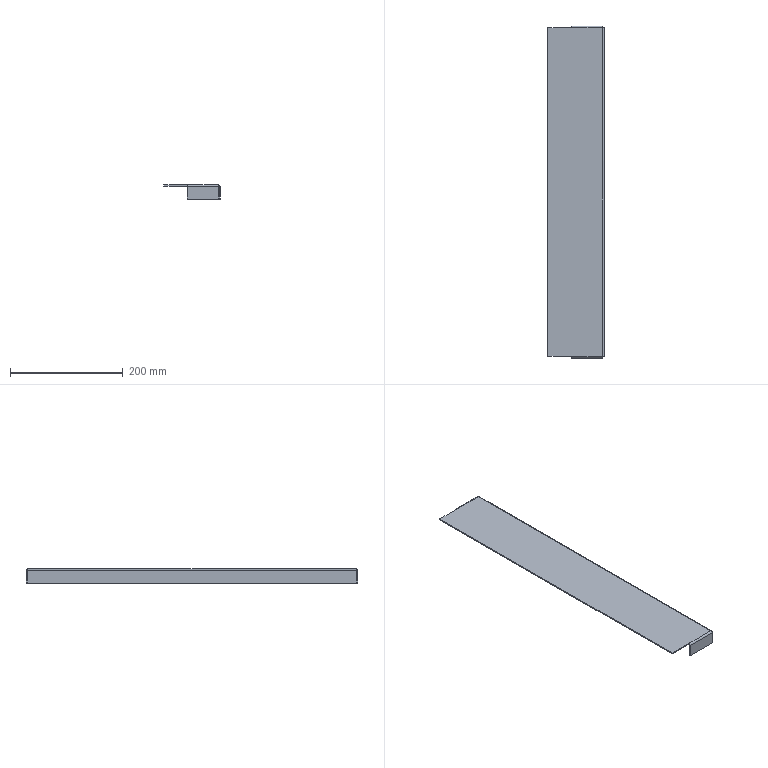Component | SolidWorks | FrontUpperAndLowerSill-1 | 1 solid | 30 faces | box 100 x 590 x 25 mm | volume 148354 mm3 | plane 20 | cylinder 6 | spline 4 | commonest cylinder face diameters 6 x3 2 x3
STEP:
#1=CARTESIAN_POINT('',(-34.876,-6.402,13.701));
#2=VERTEX_POINT('',#1);
#3=CARTESIAN_POINT('',(-32.711,-6.402,13.701));
#4=VERTEX_POINT('',#3);
#5=CARTESIAN_POINT('',(-36.529,-6.402,13.701));
#6=DIRECTION('',(1.,-0.,-0.));
#7=VECTOR('',#6,39.37);
#8=LINE('',#5,#7);
#9=EDGE_CURVE('',#2,#4,#8,.T.);
#10=ORIENTED_EDGE('',*,*,#9,.F.);
#11=CARTESIAN_POINT('',(-34.876,-6.52,13.583));
#12=VERTEX_POINT('',#11);
#13=CARTESIAN_POINT('',(-34.876,-6.402,13.583));
#14=DIRECTION('',(1.,-0.,-0.));
#15=DIRECTION('',(0.,0.,-1.));
#16=AXIS2_PLACEMENT_3D('',#13,#14,#15);
#17=CIRCLE('',#16,0.1181);
#18=EDGE_CURVE('',#2,#12,#17,.T.);
#19=ORIENTED_EDGE('',*,*,#18,.T.);
#20=CARTESIAN_POINT('',(-32.677,-6.52,13.583));
#21=VERTEX_POINT('',#20);
#22=CARTESIAN_POINT('',(-32.592,-6.52,13.583));
#23=DIRECTION('',(1.,-0.,-0.));
#24=VECTOR('',#23,39.37);
#25=LINE('',#22,#24);
#26=EDGE_CURVE('',#12,#21,#25,.T.);
#27=ORIENTED_EDGE('',*,*,#26,.T.);
#28=CARTESIAN_POINT('',(-32.711,-6.402,13.701));
#29=CARTESIAN_POINT('',(-32.709,-6.41,13.701));
#30=CARTESIAN_POINT('',(-32.708,-6.417,13.7));
#31=CARTESIAN_POINT('',(-32.705,-6.432,13.697));
#32=CARTESIAN_POINT('',(-32.704,-6.44,13.695));
#33=CARTESIAN_POINT('',(-32.701,-6.454,13.689));
#34=CARTESIAN_POINT('',(-32.699,-6.461,13.685));
#35=CARTESIAN_POINT('',(-32.696,-6.474,13.677));
#36=CARTESIAN_POINT('',(-32.695,-6.48,13.672));
#37=CARTESIAN_POINT('',(-32.692,-6.491,13.661));
#38=CARTESIAN_POINT('',(-32.691,-6.496,13.655));
#39=CARTESIAN_POINT('',(-32.688,-6.504,13.642));
#40=CARTESIAN_POINT('',(-32.687,-6.508,13.635));
#41=CARTESIAN_POINT('',(-32.682,-6.517,13.614));
#42=CARTESIAN_POINT('',(-32.68,-6.52,13.598));
#43=CARTESIAN_POINT('',(-32.677,-6.52,13.583));
#44=B_SPLINE_CURVE_WITH_KNOTS('',3,(#28,#29,#30,#31,#32,#33,#34,#35,#36,#37,#38,#39,#40,#41,#42,#43),.UNSPECIFIED.,.F.,.F.,(4,2,2,2,2,2,2,4),(0.,0.0005957,0.001191,0.001787,0.002383,0.002978,0.003574,0.004766),.UNSPECIFIED.);
#45=EDGE_CURVE('',#4,#21,#44,.T.);
#46=ORIENTED_EDGE('',*,*,#45,.F.);
#47=EDGE_LOOP('',(#10,#19,#27,#46));
#48=FACE_OUTER_BOUND('',#47,.T.);
#49=CARTESIAN_POINT('',(-36.529,-6.402,13.583));
#50=DIRECTION('',(-1.,0.,0.));
#51=DIRECTION('',(0.,-1.,-0.));
#52=AXIS2_PLACEMENT_3D('',#49,#50,#51);
#53=CYLINDRICAL_SURFACE('',#52,0.1181);
#54=ADVANCED_FACE('',(#48),#53,.T.);
#55=CARTESIAN_POINT('',(-34.876,-6.402,13.622));
#56=VERTEX_POINT('',#55);
#57=CARTESIAN_POINT('',(-34.876,-6.441,13.583));
#58=VERTEX_POINT('',#57);
#59=CARTESIAN_POINT('',(-34.876,-6.402,13.583));
#60=DIRECTION('',(1.,-0.,-0.));
#61=DIRECTION('',(0.,0.,-1.));
#62=AXIS2_PLACEMENT_3D('',#59,#60,#61);
#63=CIRCLE('',#62,0.03937);
#64=EDGE_CURVE('',#56,#58,#63,.T.);
#65=ORIENTED_EDGE('',*,*,#64,.F.);
#66=CARTESIAN_POINT('',(-32.711,-6.402,13.622));
#67=VERTEX_POINT('',#66);
#68=CARTESIAN_POINT('',(-36.529,-6.402,13.622));
#69=DIRECTION('',(1.,-0.,-0.));
#70=VECTOR('',#69,39.37);
#71=LINE('',#68,#70);
#72=EDGE_CURVE('',#56,#67,#71,.T.);
#73=ORIENTED_EDGE('',*,*,#72,.T.);
#74=CARTESIAN_POINT('',(-32.677,-6.441,13.583));
#75=VERTEX_POINT('',#74);
#76=CARTESIAN_POINT('',(-32.711,-6.402,13.622));
#77=CARTESIAN_POINT('',(-32.708,-6.407,13.622));
#78=CARTESIAN_POINT('',(-32.705,-6.412,13.621));
#79=CARTESIAN_POINT('',(-32.699,-6.422,13.617));
#80=CARTESIAN_POINT('',(-32.696,-6.426,13.614));
#81=CARTESIAN_POINT('',(-32.691,-6.433,13.607));
#82=CARTESIAN_POINT('',(-32.688,-6.436,13.603));
#83=CARTESIAN_POINT('',(-32.682,-6.44,13.593));
#84=CARTESIAN_POINT('',(-32.68,-6.441,13.588));
#85=CARTESIAN_POINT('',(-32.677,-6.441,13.583));
#86=B_SPLINE_CURVE_WITH_KNOTS('',3,(#76,#77,#78,#79,#80,#81,#82,#83,#84,#85),.UNSPECIFIED.,.F.,.F.,(4,2,2,2,4),(0.,0.0004433,0.0008867,0.00133,0.001773),.UNSPECIFIED.);
#87=EDGE_CURVE('',#67,#75,#86,.T.);
#88=ORIENTED_EDGE('',*,*,#87,.T.);
#89=CARTESIAN_POINT('',(-32.592,-6.441,13.583));
#90=DIRECTION('',(-1.,0.,0.));
#91=VECTOR('',#90,39.37);
#92=LINE('',#89,#91);
#93=EDGE_CURVE('',#75,#58,#92,.T.);
#94=ORIENTED_EDGE('',*,*,#93,.T.);
#95=EDGE_LOOP('',(#65,#73,#88,#94));
#96=FACE_OUTER_BOUND('',#95,.T.);
#97=CARTESIAN_POINT('',(-36.529,-6.402,13.583));
#98=DIRECTION('',(-1.,0.,0.));
#99=DIRECTION('',(0.,-1.,0.));
#100=AXIS2_PLACEMENT_3D('',#97,#98,#99);
#101=CYLINDRICAL_SURFACE('',#100,0.03937);
#102=ADVANCED_FACE('',(#96),#101,.F.);
#103=CARTESIAN_POINT('',(-34.876,-6.52,12.717));
#104=VERTEX_POINT('',#103);
#105=CARTESIAN_POINT('',(-34.876,-6.52,13.701));
#106=DIRECTION('',(0.,-0.,1.));
#107=VECTOR('',#106,39.37);
#108=LINE('',#105,#107);
#109=EDGE_CURVE('',#104,#12,#108,.T.);
#110=ORIENTED_EDGE('',*,*,#109,.F.);
#111=CARTESIAN_POINT('',(-32.677,-6.52,12.717));
#112=VERTEX_POINT('',#111);
#113=CARTESIAN_POINT('',(-32.592,-6.52,12.717));
#114=DIRECTION('',(-1.,0.,0.));
#115=VECTOR('',#114,39.37);
#116=LINE('',#113,#115);
#117=EDGE_CURVE('',#112,#104,#116,.T.);
#118=ORIENTED_EDGE('',*,*,#117,.F.);
#119=CARTESIAN_POINT('',(-32.677,-6.52,13.622));
#120=DIRECTION('',(0.,0.,-1.));
#121=VECTOR('',#120,39.37);
#122=LINE('',#119,#121);
#123=EDGE_CURVE('',#21,#112,#122,.T.);
#124=ORIENTED_EDGE('',*,*,#123,.F.);
#125=ORIENTED_EDGE('',*,*,#26,.F.);
#126=EDGE_LOOP('',(#110,#118,#124,#125));
#127=FACE_OUTER_BOUND('',#126,.T.);
#128=CARTESIAN_POINT('',(-32.592,-6.52,12.717));
#129=DIRECTION('',(0.,1.,0.));
#130=DIRECTION('',(0.,-0.,1.));
#131=AXIS2_PLACEMENT_3D('',#128,#129,#130);
#132=PLANE('',#131);
#133=ADVANCED_FACE('',(#127),#132,.F.);
#134=CARTESIAN_POINT('',(-32.677,-6.441,12.717));
#135=VERTEX_POINT('',#134);
#136=CARTESIAN_POINT('',(-34.876,-6.441,12.717));
#137=VERTEX_POINT('',#136);
#138=CARTESIAN_POINT('',(-32.592,-6.441,12.717));
#139=DIRECTION('',(-1.,0.,0.));
#140=VECTOR('',#139,39.37);
#141=LINE('',#138,#140);
#142=EDGE_CURVE('',#135,#137,#141,.T.);
#143=ORIENTED_EDGE('',*,*,#142,.T.);
#144=CARTESIAN_POINT('',(-34.876,-6.441,12.717));
#145=DIRECTION('',(0.,-0.,1.));
#146=VECTOR('',#145,39.37);
#147=LINE('',#144,#146);
#148=EDGE_CURVE('',#137,#58,#147,.T.);
#149=ORIENTED_EDGE('',*,*,#148,.T.);
#150=ORIENTED_EDGE('',*,*,#93,.F.);
#151=CARTESIAN_POINT('',(-32.677,-6.441,12.717));
#152=DIRECTION('',(0.,0.,-1.));
#153=VECTOR('',#152,39.37);
#154=LINE('',#151,#153);
#155=EDGE_CURVE('',#75,#135,#154,.T.);
#156=ORIENTED_EDGE('',*,*,#155,.T.);
#157=EDGE_LOOP('',(#143,#149,#150,#156));
#158=FACE_OUTER_BOUND('',#157,.T.);
#159=CARTESIAN_POINT('',(-32.592,-6.441,12.717));
#160=DIRECTION('',(0.,1.,0.));
#161=DIRECTION('',(0.,-0.,1.));
#162=AXIS2_PLACEMENT_3D('',#159,#160,#161);
#163=PLANE('',#162);
#164=ADVANCED_FACE('',(#158),#163,.T.);
#165=ORIENTED_EDGE('',*,*,#117,.T.);
#166=CARTESIAN_POINT('',(-34.876,-6.402,12.717));
#167=DIRECTION('',(-0.,-1.,-0.));
#168=VECTOR('',#167,39.37);
#169=LINE('',#166,#168);
#170=EDGE_CURVE('',#137,#104,#169,.T.);
#171=ORIENTED_EDGE('',*,*,#170,.F.);
#172=ORIENTED_EDGE('',*,*,#142,.F.);
#173=CARTESIAN_POINT('',(-32.677,-6.52,12.717));
#174=DIRECTION('',(-0.,-1.,-0.));
#175=VECTOR('',#174,39.37);
#176=LINE('',#173,#175);
#177=EDGE_CURVE('',#135,#112,#176,.T.);
#178=ORIENTED_EDGE('',*,*,#177,.T.);
#179=EDGE_LOOP('',(#165,#171,#172,#178));
#180=FACE_OUTER_BOUND('',#179,.T.);
#181=CARTESIAN_POINT('',(-32.592,-6.52,12.717));
#182=DIRECTION('',(-0.,0.,-1.));
#183=DIRECTION('',(0.,1.,0.));
#184=AXIS2_PLACEMENT_3D('',#181,#182,#183);
#185=PLANE('',#184);
#186=ADVANCED_FACE('',(#180),#185,.T.);
#187=CARTESIAN_POINT('',(-32.711,16.59,13.622));
#188=VERTEX_POINT('',#187);
#189=CARTESIAN_POINT('',(-32.711,-6.436,13.622));
#190=DIRECTION('',(0.,1.,0.));
#191=VECTOR('',#190,39.37);
#192=LINE('',#189,#191);
#193=EDGE_CURVE('',#67,#188,#192,.T.);
#194=ORIENTED_EDGE('',*,*,#193,.F.);
#195=ORIENTED_EDGE('',*,*,#72,.F.);
#196=CARTESIAN_POINT('',(-36.529,-6.402,13.622));
#197=VERTEX_POINT('',#196);
#198=CARTESIAN_POINT('',(-36.529,-6.402,13.622));
#199=DIRECTION('',(1.,-0.,-0.));
#200=VECTOR('',#199,39.37);
#201=LINE('',#198,#200);
#202=EDGE_CURVE('',#197,#56,#201,.T.);
#203=ORIENTED_EDGE('',*,*,#202,.F.);
#204=CARTESIAN_POINT('',(-36.529,16.59,13.622));
#205=VERTEX_POINT('',#204);
#206=CARTESIAN_POINT('',(-36.529,16.708,13.622));
#207=DIRECTION('',(-0.,-1.,-0.));
#208=VECTOR('',#207,39.37);
#209=LINE('',#206,#208);
#210=EDGE_CURVE('',#205,#197,#209,.T.);
#211=ORIENTED_EDGE('',*,*,#210,.F.);
#212=CARTESIAN_POINT('',(-34.876,16.59,13.622));
#213=VERTEX_POINT('',#212);
#214=CARTESIAN_POINT('',(-32.677,16.59,13.622));
#215=DIRECTION('',(-1.,0.,0.));
#216=VECTOR('',#215,39.37);
#217=LINE('',#214,#216);
#218=EDGE_CURVE('',#213,#205,#217,.T.);
#219=ORIENTED_EDGE('',*,*,#218,.F.);
#220=CARTESIAN_POINT('',(-32.677,16.59,13.622));
#221=DIRECTION('',(-1.,0.,0.));
#222=VECTOR('',#221,39.37);
#223=LINE('',#220,#222);
#224=EDGE_CURVE('',#188,#213,#223,.T.);
#225=ORIENTED_EDGE('',*,*,#224,.F.);
#226=EDGE_LOOP('',(#194,#195,#203,#211,#219,#225));
#227=FACE_OUTER_BOUND('',#226,.T.);
#228=CARTESIAN_POINT('',(-36.529,-6.52,13.622));
#229=DIRECTION('',(0.,-0.,1.));
#230=DIRECTION('',(-0.,-1.,-0.));
#231=AXIS2_PLACEMENT_3D('',#228,#229,#230);
#232=PLANE('',#231);
#233=ADVANCED_FACE('',(#227),#232,.F.);
#234=CARTESIAN_POINT('',(-36.529,-6.402,13.701));
#235=VERTEX_POINT('',#234);
#236=CARTESIAN_POINT('',(-36.529,-6.402,13.701));
#237=DIRECTION('',(1.,-0.,-0.));
#238=VECTOR('',#237,39.37);
#239=LINE('',#236,#238);
#240=EDGE_CURVE('',#235,#2,#239,.T.);
#241=ORIENTED_EDGE('',*,*,#240,.T.);
#242=ORIENTED_EDGE('',*,*,#9,.T.);
#243=CARTESIAN_POINT('',(-32.711,16.59,13.701));
#244=VERTEX_POINT('',#243);
#245=CARTESIAN_POINT('',(-32.711,-6.436,13.701));
#246=DIRECTION('',(0.,1.,0.));
#247=VECTOR('',#246,39.37);
#248=LINE('',#245,#247);
#249=EDGE_CURVE('',#4,#244,#248,.T.);
#250=ORIENTED_EDGE('',*,*,#249,.T.);
#251=CARTESIAN_POINT('',(-34.876,16.59,13.701));
#252=VERTEX_POINT('',#251);
#253=CARTESIAN_POINT('',(-32.677,16.59,13.701));
#254=DIRECTION('',(-1.,0.,0.));
#255=VECTOR('',#254,39.37);
#256=LINE('',#253,#255);
#257=EDGE_CURVE('',#244,#252,#256,.T.);
#258=ORIENTED_EDGE('',*,*,#257,.T.);
#259=CARTESIAN_POINT('',(-36.529,16.59,13.701));
#260=VERTEX_POINT('',#259);
#261=CARTESIAN_POINT('',(-34.876,16.59,13.701));
#262=DIRECTION('',(-1.,0.,0.));
#263=VECTOR('',#262,39.37);
#264=LINE('',#261,#263);
#265=EDGE_CURVE('',#252,#260,#264,.T.);
#266=ORIENTED_EDGE('',*,*,#265,.T.);
#267=CARTESIAN_POINT('',(-36.529,16.708,13.701));
#268=DIRECTION('',(-0.,-1.,-0.));
#269=VECTOR('',#268,39.37);
#270=LINE('',#267,#269);
#271=EDGE_CURVE('',#260,#235,#270,.T.);
#272=ORIENTED_EDGE('',*,*,#271,.T.);
#273=EDGE_LOOP('',(#241,#242,#250,#258,#266,#272));
#274=FACE_OUTER_BOUND('',#273,.T.);
#275=CARTESIAN_POINT('',(-36.529,-6.52,13.701));
#276=DIRECTION('',(0.,-0.,1.));
#277=DIRECTION('',(-0.,-1.,-0.));
#278=AXIS2_PLACEMENT_3D('',#275,#276,#277);
#279=PLANE('',#278);
#280=ADVANCED_FACE('',(#274),#279,.T.);
#281=ORIENTED_EDGE('',*,*,#210,.T.);
#282=CARTESIAN_POINT('',(-36.529,-6.402,13.622));
#283=DIRECTION('',(0.,-0.,1.));
#284=VECTOR('',#283,39.37);
#285=LINE('',#282,#284);
#286=EDGE_CURVE('',#197,#235,#285,.T.);
#287=ORIENTED_EDGE('',*,*,#286,.T.);
#288=ORIENTED_EDGE('',*,*,#271,.F.);
#289=CARTESIAN_POINT('',(-36.529,16.59,13.622));
#290=DIRECTION('',(0.,-0.,1.));
#291=VECTOR('',#290,39.37);
#292=LINE('',#289,#291);
#293=EDGE_CURVE('',#205,#260,#292,.T.);
#294=ORIENTED_EDGE('',*,*,#293,.F.);
#295=EDGE_LOOP('',(#281,#287,#288,#294));
#296=FACE_OUTER_BOUND('',#295,.T.);
#297=CARTESIAN_POINT('',(-36.529,16.708,13.622));
#298=DIRECTION('',(-1.,0.,0.));
#299=DIRECTION('',(-0.,0.,-1.));
#300=AXIS2_PLACEMENT_3D('',#297,#298,#299);
#301=PLANE('',#300);
#302=ADVANCED_FACE('',(#296),#301,.T.);
#303=CARTESIAN_POINT('',(-32.677,16.63,13.583));
#304=VERTEX_POINT('',#303);
#305=CARTESIAN_POINT('',(-32.677,16.63,13.583));
#306=CARTESIAN_POINT('',(-32.68,16.63,13.588));
#307=CARTESIAN_POINT('',(-32.682,16.629,13.593));
#308=CARTESIAN_POINT('',(-32.688,16.625,13.602));
#309=CARTESIAN_POINT('',(-32.691,16.622,13.607));
#310=CARTESIAN_POINT('',(-32.696,16.615,13.614));
#311=CARTESIAN_POINT('',(-32.699,16.61,13.617));
#312=CARTESIAN_POINT('',(-32.705,16.601,13.621));
#313=CARTESIAN_POINT('',(-32.708,16.596,13.622));
#314=CARTESIAN_POINT('',(-32.711,16.59,13.622));
#315=B_SPLINE_CURVE_WITH_KNOTS('',3,(#305,#306,#307,#308,#309,#310,#311,#312,#313,#314),.UNSPECIFIED.,.F.,.F.,(4,2,2,2,4),(0.,0.0004433,0.0008867,0.00133,0.001773),.UNSPECIFIED.);
#316=EDGE_CURVE('',#304,#188,#315,.T.);
#317=ORIENTED_EDGE('',*,*,#316,.F.);
#318=CARTESIAN_POINT('',(-32.677,16.708,13.583));
#319=VERTEX_POINT('',#318);
#320=CARTESIAN_POINT('',(-32.677,16.63,13.583));
#321=DIRECTION('',(-0.,-1.,-0.));
#322=VECTOR('',#321,39.37);
#323=LINE('',#320,#322);
#324=EDGE_CURVE('',#319,#304,#323,.T.);
#325=ORIENTED_EDGE('',*,*,#324,.F.);
#326=CARTESIAN_POINT('',(-32.677,16.708,13.583));
#327=CARTESIAN_POINT('',(-32.678,16.708,13.59));
#328=CARTESIAN_POINT('',(-32.68,16.708,13.598));
#329=CARTESIAN_POINT('',(-32.682,16.705,13.613));
#330=CARTESIAN_POINT('',(-32.684,16.702,13.621));
#331=CARTESIAN_POINT('',(-32.687,16.697,13.635));
#332=CARTESIAN_POINT('',(-32.688,16.693,13.642));
#333=CARTESIAN_POINT('',(-32.691,16.684,13.655));
#334=CARTESIAN_POINT('',(-32.692,16.679,13.661));
#335=CARTESIAN_POINT('',(-32.695,16.668,13.672));
#336=CARTESIAN_POINT('',(-32.696,16.663,13.677));
#337=CARTESIAN_POINT('',(-32.699,16.65,13.685));
#338=CARTESIAN_POINT('',(-32.701,16.643,13.689));
#339=CARTESIAN_POINT('',(-32.705,16.621,13.698));
#340=CARTESIAN_POINT('',(-32.708,16.606,13.701));
#341=CARTESIAN_POINT('',(-32.711,16.59,13.701));
#342=B_SPLINE_CURVE_WITH_KNOTS('',3,(#326,#327,#328,#329,#330,#331,#332,#333,#334,#335,#336,#337,#338,#339,#340,#341),.UNSPECIFIED.,.F.,.F.,(4,2,2,2,2,2,2,4),(0.,0.0005957,0.001191,0.001787,0.002383,0.002978,0.003574,0.004766),.UNSPECIFIED.);
#343=EDGE_CURVE('',#319,#244,#342,.T.);
#344=ORIENTED_EDGE('',*,*,#343,.T.);
#345=CARTESIAN_POINT('',(-32.711,16.59,13.622));
#346=DIRECTION('',(0.,-0.,1.));
#347=VECTOR('',#346,39.37);
#348=LINE('',#345,#347);
#349=EDGE_CURVE('',#188,#244,#348,.T.);
#350=ORIENTED_EDGE('',*,*,#349,.F.);
#351=EDGE_LOOP('',(#317,#325,#344,#350));
#352=FACE_OUTER_BOUND('',#351,.T.);
#353=CARTESIAN_POINT('',(-32.677,16.709,13.583));
#354=CARTESIAN_POINT('',(-32.68,16.709,13.598));
#355=CARTESIAN_POINT('',(-32.682,16.706,13.614));
#356=CARTESIAN_POINT('',(-32.688,16.694,13.643));
#357=CARTESIAN_POINT('',(-32.691,16.685,13.656));
#358=CARTESIAN_POINT('',(-32.696,16.663,13.678));
#359=CARTESIAN_POINT('',(-32.699,16.65,13.687));
#360=CARTESIAN_POINT('',(-32.705,16.621,13.698));
#361=CARTESIAN_POINT('',(-32.708,16.606,13.702));
#362=CARTESIAN_POINT('',(-32.711,16.59,13.702));
#363=CARTESIAN_POINT('',(-32.677,16.708,13.583));
#364=CARTESIAN_POINT('',(-32.68,16.708,13.598));
#365=CARTESIAN_POINT('',(-32.682,16.705,13.614));
#366=CARTESIAN_POINT('',(-32.688,16.694,13.642));
#367=CARTESIAN_POINT('',(-32.691,16.685,13.655));
#368=CARTESIAN_POINT('',(-32.696,16.663,13.677));
#369=CARTESIAN_POINT('',(-32.699,16.65,13.686));
#370=CARTESIAN_POINT('',(-32.705,16.621,13.698));
#371=CARTESIAN_POINT('',(-32.708,16.606,13.701));
#372=CARTESIAN_POINT('',(-32.711,16.59,13.701));
#373=CARTESIAN_POINT('',(-32.677,16.63,13.583));
#374=CARTESIAN_POINT('',(-32.68,16.63,13.588));
#375=CARTESIAN_POINT('',(-32.682,16.629,13.593));
#376=CARTESIAN_POINT('',(-32.688,16.625,13.603));
#377=CARTESIAN_POINT('',(-32.691,16.622,13.607));
#378=CARTESIAN_POINT('',(-32.696,16.615,13.614));
#379=CARTESIAN_POINT('',(-32.699,16.61,13.617));
#380=CARTESIAN_POINT('',(-32.705,16.601,13.621));
#381=CARTESIAN_POINT('',(-32.708,16.596,13.622));
#382=CARTESIAN_POINT('',(-32.711,16.59,13.622));
#383=CARTESIAN_POINT('',(-32.677,16.629,13.583));
#384=CARTESIAN_POINT('',(-32.68,16.629,13.588));
#385=CARTESIAN_POINT('',(-32.682,16.628,13.593));
#386=CARTESIAN_POINT('',(-32.688,16.624,13.602));
#387=CARTESIAN_POINT('',(-32.691,16.621,13.606));
#388=CARTESIAN_POINT('',(-32.696,16.614,13.614));
#389=CARTESIAN_POINT('',(-32.699,16.61,13.616));
#390=CARTESIAN_POINT('',(-32.705,16.6,13.62));
#391=CARTESIAN_POINT('',(-32.708,16.595,13.621));
#392=CARTESIAN_POINT('',(-32.711,16.59,13.621));
#393=B_SPLINE_SURFACE_WITH_KNOTS('',1,3,((#353,#354,#355,#356,#357,#358,#359,#360,#361,#362),(#363,#364,#365,#366,#367,#368,#369,#370,#371,#372),(#373,#374,#375,#376,#377,#378,#379,#380,#381,#382),(#383,#384,#385,#386,#387,#388,#389,#390,#391,#392)),.UNSPECIFIED.,.F.,.F.,.F.,(2,1,1,2),(4,2,2,2,4),(-0.01,0.,1.,1.01),(0.,0.25,0.5,0.75,1.),.UNSPECIFIED.);
#394=ADVANCED_FACE('',(#352),#393,.F.);
#395=CARTESIAN_POINT('',(-34.876,16.708,13.583));
#396=VERTEX_POINT('',#395);
#397=CARTESIAN_POINT('',(-34.876,16.59,13.583));
#398=DIRECTION('',(-1.,0.,0.));
#399=DIRECTION('',(0.,0.,1.));
#400=AXIS2_PLACEMENT_3D('',#397,#398,#399);
#401=CIRCLE('',#400,0.1181);
#402=EDGE_CURVE('',#252,#396,#401,.T.);
#403=ORIENTED_EDGE('',*,*,#402,.F.);
#404=ORIENTED_EDGE('',*,*,#257,.F.);
#405=ORIENTED_EDGE('',*,*,#343,.F.);
#406=CARTESIAN_POINT('',(-32.592,16.708,13.583));
#407=DIRECTION('',(1.,-0.,-0.));
#408=VECTOR('',#407,39.37);
#409=LINE('',#406,#408);
#410=EDGE_CURVE('',#396,#319,#409,.T.);
#411=ORIENTED_EDGE('',*,*,#410,.F.);
#412=EDGE_LOOP('',(#403,#404,#405,#411));
#413=FACE_OUTER_BOUND('',#412,.T.);
#414=CARTESIAN_POINT('',(-32.677,16.59,13.583));
#415=DIRECTION('',(1.,-0.,-0.));
#416=DIRECTION('',(0.,1.,0.));
#417=AXIS2_PLACEMENT_3D('',#414,#415,#416);
#418=CYLINDRICAL_SURFACE('',#417,0.1181);
#419=ADVANCED_FACE('',(#413),#418,.T.);
#420=ORIENTED_EDGE('',*,*,#224,.T.);
#421=CARTESIAN_POINT('',(-34.876,16.63,13.583));
#422=VERTEX_POINT('',#421);
#423=CARTESIAN_POINT('',(-34.876,16.59,13.583));
#424=DIRECTION('',(-1.,0.,0.));
#425=DIRECTION('',(0.,0.,1.));
#426=AXIS2_PLACEMENT_3D('',#423,#424,#425);
#427=CIRCLE('',#426,0.03937);
#428=EDGE_CURVE('',#213,#422,#427,.T.);
#429=ORIENTED_EDGE('',*,*,#428,.T.);
#430=CARTESIAN_POINT('',(-36.529,16.63,13.583));
#431=DIRECTION('',(1.,-0.,-0.));
#432=VECTOR('',#431,39.37);
#433=LINE('',#430,#432);
#434=EDGE_CURVE('',#422,#304,#433,.T.);
#435=ORIENTED_EDGE('',*,*,#434,.T.);
#436=ORIENTED_EDGE('',*,*,#316,.T.);
#437=EDGE_LOOP('',(#420,#429,#435,#436));
#438=FACE_OUTER_BOUND('',#437,.T.);
#439=CARTESIAN_POINT('',(-32.677,16.59,13.583));
#440=DIRECTION('',(1.,-0.,-0.));
#441=DIRECTION('',(0.,1.,0.));
#442=AXIS2_PLACEMENT_3D('',#439,#440,#441);
#443=CYLINDRICAL_SURFACE('',#442,0.03937);
#444=ADVANCED_FACE('',(#438),#443,.F.);
#445=CARTESIAN_POINT('',(-34.876,16.708,12.717));
#446=VERTEX_POINT('',#445);
#447=CARTESIAN_POINT('',(-34.876,16.708,13.701));
#448=DIRECTION('',(-0.,0.,-1.));
#449=VECTOR('',#448,39.37);
#450=LINE('',#447,#449);
#451=EDGE_CURVE('',#396,#446,#450,.T.);
#452=ORIENTED_EDGE('',*,*,#451,.F.);
#453=ORIENTED_EDGE('',*,*,#410,.T.);
#454=CARTESIAN_POINT('',(-32.677,16.708,12.717));
#455=VERTEX_POINT('',#454);
#456=CARTESIAN_POINT('',(-32.677,16.708,13.622));
#457=DIRECTION('',(-0.,-0.,1.));
#458=VECTOR('',#457,39.37);
#459=LINE('',#456,#458);
#460=EDGE_CURVE('',#455,#319,#459,.T.);
#461=ORIENTED_EDGE('',*,*,#460,.F.);
#462=CARTESIAN_POINT('',(-32.592,16.708,12.717));
#463=DIRECTION('',(1.,-0.,-0.));
#464=VECTOR('',#463,39.37);
#465=LINE('',#462,#464);
#466=EDGE_CURVE('',#446,#455,#465,.T.);
#467=ORIENTED_EDGE('',*,*,#466,.F.);
#468=EDGE_LOOP('',(#452,#453,#461,#467));
#469=FACE_OUTER_BOUND('',#468,.T.);
#470=CARTESIAN_POINT('',(-32.592,16.708,13.622));
#471=DIRECTION('',(0.,1.,0.));
#472=DIRECTION('',(0.,-0.,1.));
#473=AXIS2_PLACEMENT_3D('',#470,#471,#472);
#474=PLANE('',#473);
#475=ADVANCED_FACE('',(#469),#474,.T.);
#476=ORIENTED_EDGE('',*,*,#434,.F.);
#477=CARTESIAN_POINT('',(-34.876,16.63,12.717));
#478=VERTEX_POINT('',#477);
#479=CARTESIAN_POINT('',(-34.876,16.63,13.622));
#480=DIRECTION('',(-0.,0.,-1.));
#481=VECTOR('',#480,39.37);
#482=LINE('',#479,#481);
#483=EDGE_CURVE('',#422,#478,#482,.T.);
#484=ORIENTED_EDGE('',*,*,#483,.T.);
#485=CARTESIAN_POINT('',(-32.677,16.63,12.717));
#486=VERTEX_POINT('',#485);
#487=CARTESIAN_POINT('',(-32.592,16.63,12.717));
#488=DIRECTION('',(1.,-0.,-0.));
#489=VECTOR('',#488,39.37);
#490=LINE('',#487,#489);
#491=EDGE_CURVE('',#478,#486,#490,.T.);
#492=ORIENTED_EDGE('',*,*,#491,.T.);
#493=CARTESIAN_POINT('',(-32.677,16.63,13.622));
#494=DIRECTION('',(0.,0.,-1.));
#495=VECTOR('',#494,39.37);
#496=LINE('',#493,#495);
#497=EDGE_CURVE('',#304,#486,#496,.T.);
#498=ORIENTED_EDGE('',*,*,#497,.F.);
#499=EDGE_LOOP('',(#476,#484,#492,#498));
#500=FACE_OUTER_BOUND('',#499,.T.);
#501=CARTESIAN_POINT('',(-32.592,16.63,13.622));
#502=DIRECTION('',(0.,1.,0.));
#503=DIRECTION('',(0.,-0.,1.));
#504=AXIS2_PLACEMENT_3D('',#501,#502,#503);
#505=PLANE('',#504);
#506=ADVANCED_FACE('',(#500),#505,.F.);
#507=CARTESIAN_POINT('',(-34.876,16.59,12.717));
#508=DIRECTION('',(-0.,-1.,-0.));
#509=VECTOR('',#508,39.37);
#510=LINE('',#507,#509);
#511=EDGE_CURVE('',#446,#478,#510,.T.);
#512=ORIENTED_EDGE('',*,*,#511,.F.);
#513=ORIENTED_EDGE('',*,*,#466,.T.);
#514=CARTESIAN_POINT('',(-32.677,16.63,12.717));
#515=DIRECTION('',(0.,1.,0.));
#516=VECTOR('',#515,39.37);
#517=LINE('',#514,#516);
#518=EDGE_CURVE('',#486,#455,#517,.T.);
#519=ORIENTED_EDGE('',*,*,#518,.F.);
#520=ORIENTED_EDGE('',*,*,#491,.F.);
#521=EDGE_LOOP('',(#512,#513,#519,#520));
#522=FACE_OUTER_BOUND('',#521,.T.);
#523=CARTESIAN_POINT('',(-32.592,16.708,12.717));
#524=DIRECTION('',(-0.,0.,-1.));
#525=DIRECTION('',(0.,1.,0.));
#526=AXIS2_PLACEMENT_3D('',#523,#524,#525);
#527=PLANE('',#526);
#528=ADVANCED_FACE('',(#522),#527,.T.);
#529=ORIENTED_EDGE('',*,*,#497,.T.);
#530=ORIENTED_EDGE('',*,*,#518,.T.);
#531=ORIENTED_EDGE('',*,*,#460,.T.);
#532=ORIENTED_EDGE('',*,*,#324,.T.);
#533=EDGE_LOOP('',(#529,#530,#531,#532));
#534=FACE_OUTER_BOUND('',#533,.T.);
#535=CARTESIAN_POINT('',(-32.677,16.63,13.622));
#536=DIRECTION('',(-1.,0.,-0.));
#537=DIRECTION('',(0.,0.,-1.));
#538=AXIS2_PLACEMENT_3D('',#535,#536,#537);
#539=PLANE('',#538);
#540=ADVANCED_FACE('',(#534),#539,.F.);
#541=CARTESIAN_POINT('',(-32.677,-6.441,13.583));
#542=DIRECTION('',(0.,1.,0.));
#543=VECTOR('',#542,39.37);
#544=LINE('',#541,#543);
#545=EDGE_CURVE('',#21,#75,#544,.T.);
#546=ORIENTED_EDGE('',*,*,#545,.T.);
#547=ORIENTED_EDGE('',*,*,#87,.F.);
#548=CARTESIAN_POINT('',(-32.711,-6.402,13.622));
#549=DIRECTION('',(0.,-0.,1.));
#550=VECTOR('',#549,39.37);
#551=LINE('',#548,#550);
#552=EDGE_CURVE('',#67,#4,#551,.T.);
#553=ORIENTED_EDGE('',*,*,#552,.T.);
#554=ORIENTED_EDGE('',*,*,#45,.T.);
#555=EDGE_LOOP('',(#546,#547,#553,#554));
#556=FACE_OUTER_BOUND('',#555,.T.);
#557=CARTESIAN_POINT('',(-32.711,-6.402,13.702));
#558=CARTESIAN_POINT('',(-32.708,-6.417,13.702));
#559=CARTESIAN_POINT('',(-32.705,-6.433,13.698));
#560=CARTESIAN_POINT('',(-32.699,-6.462,13.687));
#561=CARTESIAN_POINT('',(-32.696,-6.475,13.678));
#562=CARTESIAN_POINT('',(-32.691,-6.497,13.656));
#563=CARTESIAN_POINT('',(-32.688,-6.506,13.643));
#564=CARTESIAN_POINT('',(-32.682,-6.518,13.614));
#565=CARTESIAN_POINT('',(-32.68,-6.521,13.598));
#566=CARTESIAN_POINT('',(-32.677,-6.521,13.583));
#567=CARTESIAN_POINT('',(-32.711,-6.402,13.701));
#568=CARTESIAN_POINT('',(-32.708,-6.417,13.701));
#569=CARTESIAN_POINT('',(-32.705,-6.433,13.698));
#570=CARTESIAN_POINT('',(-32.699,-6.461,13.686));
#571=CARTESIAN_POINT('',(-32.696,-6.474,13.677));
#572=CARTESIAN_POINT('',(-32.691,-6.496,13.655));
#573=CARTESIAN_POINT('',(-32.688,-6.505,13.642));
#574=CARTESIAN_POINT('',(-32.682,-6.517,13.614));
#575=CARTESIAN_POINT('',(-32.68,-6.52,13.598));
#576=CARTESIAN_POINT('',(-32.677,-6.52,13.583));
#577=CARTESIAN_POINT('',(-32.711,-6.402,13.622));
#578=CARTESIAN_POINT('',(-32.708,-6.407,13.622));
#579=CARTESIAN_POINT('',(-32.705,-6.412,13.621));
#580=CARTESIAN_POINT('',(-32.699,-6.422,13.617));
#581=CARTESIAN_POINT('',(-32.696,-6.426,13.614));
#582=CARTESIAN_POINT('',(-32.691,-6.433,13.607));
#583=CARTESIAN_POINT('',(-32.688,-6.436,13.603));
#584=CARTESIAN_POINT('',(-32.682,-6.44,13.593));
#585=CARTESIAN_POINT('',(-32.68,-6.441,13.588));
#586=CARTESIAN_POINT('',(-32.677,-6.441,13.583));
#587=CARTESIAN_POINT('',(-32.711,-6.402,13.621));
#588=CARTESIAN_POINT('',(-32.708,-6.407,13.621));
#589=CARTESIAN_POINT('',(-32.705,-6.412,13.62));
#590=CARTESIAN_POINT('',(-32.699,-6.421,13.616));
#591=CARTESIAN_POINT('',(-32.696,-6.425,13.614));
#592=CARTESIAN_POINT('',(-32.691,-6.433,13.606));
#593=CARTESIAN_POINT('',(-32.688,-6.435,13.602));
#594=CARTESIAN_POINT('',(-32.682,-6.439,13.593));
#595=CARTESIAN_POINT('',(-32.68,-6.44,13.588));
#596=CARTESIAN_POINT('',(-32.677,-6.44,13.583));
#597=B_SPLINE_SURFACE_WITH_KNOTS('',1,3,((#557,#558,#559,#560,#561,#562,#563,#564,#565,#566),(#567,#568,#569,#570,#571,#572,#573,#574,#575,#576),(#577,#578,#579,#580,#581,#582,#583,#584,#585,#586),(#587,#588,#589,#590,#591,#592,#593,#594,#595,#596)),.UNSPECIFIED.,.F.,.F.,.F.,(2,1,1,2),(4,2,2,2,4),(-0.01,0.,1.,1.01),(0.,0.25,0.5,0.75,1.),.UNSPECIFIED.);
#598=ADVANCED_FACE('',(#556),#597,.F.);
#599=ORIENTED_EDGE('',*,*,#177,.F.);
#600=ORIENTED_EDGE('',*,*,#155,.F.);
#601=ORIENTED_EDGE('',*,*,#545,.F.);
#602=ORIENTED_EDGE('',*,*,#123,.T.);
#603=EDGE_LOOP('',(#599,#600,#601,#602));
#604=FACE_OUTER_BOUND('',#603,.T.);
#605=CARTESIAN_POINT('',(-32.677,-6.441,13.622));
#606=DIRECTION('',(1.,-0.,0.));
#607=DIRECTION('',(-0.,-0.,1.));
#608=AXIS2_PLACEMENT_3D('',#605,#606,#607);
#609=PLANE('',#608);
#610=ADVANCED_FACE('',(#604),#609,.T.);
#611=CARTESIAN_POINT('',(-32.592,16.624,13.583));
#612=VERTEX_POINT('',#611);
#613=CARTESIAN_POINT('',(-32.671,16.624,13.583));
#614=VERTEX_POINT('',#613);
#615=CARTESIAN_POINT('',(-32.671,16.624,13.583));
#616=DIRECTION('',(-1.,0.,-0.));
#617=VECTOR('',#616,39.37);
#618=LINE('',#615,#617);
#619=EDGE_CURVE('',#612,#614,#618,.T.);
#620=ORIENTED_EDGE('',*,*,#619,.T.);
#621=CARTESIAN_POINT('',(-32.711,16.59,13.622));
#622=CARTESIAN_POINT('',(-32.705,16.593,13.622));
#623=CARTESIAN_POINT('',(-32.7,16.596,13.621));
#624=CARTESIAN_POINT('',(-32.691,16.602,13.617));
#625=CARTESIAN_POINT('',(-32.686,16.604,13.614));
#626=CARTESIAN_POINT('',(-32.679,16.61,13.607));
#627=CARTESIAN_POINT('',(-32.676,16.613,13.603));
#628=CARTESIAN_POINT('',(-32.672,16.619,13.593));
#629=CARTESIAN_POINT('',(-32.671,16.621,13.588));
#630=CARTESIAN_POINT('',(-32.671,16.624,13.583));
#631=B_SPLINE_CURVE_WITH_KNOTS('',3,(#621,#622,#623,#624,#625,#626,#627,#628,#629,#630),.UNSPECIFIED.,.F.,.F.,(4,2,2,2,4),(0.,0.0004433,0.0008867,0.00133,0.001773),.UNSPECIFIED.);
#632=EDGE_CURVE('',#188,#614,#631,.T.);
#633=ORIENTED_EDGE('',*,*,#632,.F.);
#634=ORIENTED_EDGE('',*,*,#349,.T.);
#635=CARTESIAN_POINT('',(-32.711,16.59,13.701));
#636=CARTESIAN_POINT('',(-32.703,16.592,13.701));
#637=CARTESIAN_POINT('',(-32.695,16.593,13.7));
#638=CARTESIAN_POINT('',(-32.68,16.596,13.697));
#639=CARTESIAN_POINT('',(-32.672,16.597,13.695));
#640=CARTESIAN_POINT('',(-32.658,16.6,13.689));
#641=CARTESIAN_POINT('',(-32.651,16.602,13.685));
#642=CARTESIAN_POINT('',(-32.639,16.604,13.677));
#643=CARTESIAN_POINT('',(-32.633,16.606,13.672));
#644=CARTESIAN_POINT('',(-32.622,16.609,13.661));
#645=CARTESIAN_POINT('',(-32.617,16.61,13.655));
#646=CARTESIAN_POINT('',(-32.608,16.613,13.642));
#647=CARTESIAN_POINT('',(-32.604,16.614,13.635));
#648=CARTESIAN_POINT('',(-32.596,16.618,13.614));
#649=CARTESIAN_POINT('',(-32.592,16.621,13.598));
#650=CARTESIAN_POINT('',(-32.592,16.624,13.583));
#651=B_SPLINE_CURVE_WITH_KNOTS('',3,(#635,#636,#637,#638,#639,#640,#641,#642,#643,#644,#645,#646,#647,#648,#649,#650),.UNSPECIFIED.,.F.,.F.,(4,2,2,2,2,2,2,4),(0.,0.0005957,0.001191,0.001787,0.002383,0.002978,0.003574,0.004766),.UNSPECIFIED.);
#652=EDGE_CURVE('',#244,#612,#651,.T.);
#653=ORIENTED_EDGE('',*,*,#652,.T.);
#654=EDGE_LOOP('',(#620,#633,#634,#653));
#655=FACE_OUTER_BOUND('',#654,.T.);
#656=CARTESIAN_POINT('',(-32.711,16.59,13.702));
#657=CARTESIAN_POINT('',(-32.695,16.593,13.702));
#658=CARTESIAN_POINT('',(-32.679,16.596,13.698));
#659=CARTESIAN_POINT('',(-32.651,16.602,13.687));
#660=CARTESIAN_POINT('',(-32.637,16.604,13.678));
#661=CARTESIAN_POINT('',(-32.615,16.61,13.656));
#662=CARTESIAN_POINT('',(-32.607,16.613,13.643));
#663=CARTESIAN_POINT('',(-32.595,16.619,13.614));
#664=CARTESIAN_POINT('',(-32.592,16.621,13.598));
#665=CARTESIAN_POINT('',(-32.592,16.624,13.583));
#666=CARTESIAN_POINT('',(-32.711,16.59,13.701));
#667=CARTESIAN_POINT('',(-32.695,16.593,13.701));
#668=CARTESIAN_POINT('',(-32.68,16.596,13.698));
#669=CARTESIAN_POINT('',(-32.651,16.602,13.686));
#670=CARTESIAN_POINT('',(-32.638,16.604,13.677));
#671=CARTESIAN_POINT('',(-32.616,16.61,13.655));
#672=CARTESIAN_POINT('',(-32.607,16.613,13.642));
#673=CARTESIAN_POINT('',(-32.596,16.619,13.614));
#674=CARTESIAN_POINT('',(-32.592,16.621,13.598));
#675=CARTESIAN_POINT('',(-32.592,16.624,13.583));
#676=CARTESIAN_POINT('',(-32.711,16.59,13.622));
#677=CARTESIAN_POINT('',(-32.705,16.593,13.622));
#678=CARTESIAN_POINT('',(-32.7,16.596,13.621));
#679=CARTESIAN_POINT('',(-32.691,16.602,13.617));
#680=CARTESIAN_POINT('',(-32.686,16.604,13.614));
#681=CARTESIAN_POINT('',(-32.679,16.61,13.607));
#682=CARTESIAN_POINT('',(-32.676,16.613,13.603));
#683=CARTESIAN_POINT('',(-32.672,16.619,13.593));
#684=CARTESIAN_POINT('',(-32.671,16.621,13.588));
#685=CARTESIAN_POINT('',(-32.671,16.624,13.583));
#686=CARTESIAN_POINT('',(-32.711,16.59,13.621));
#687=CARTESIAN_POINT('',(-32.705,16.593,13.621));
#688=CARTESIAN_POINT('',(-32.7,16.596,13.62));
#689=CARTESIAN_POINT('',(-32.691,16.602,13.616));
#690=CARTESIAN_POINT('',(-32.687,16.604,13.614));
#691=CARTESIAN_POINT('',(-32.68,16.61,13.606));
#692=CARTESIAN_POINT('',(-32.677,16.613,13.602));
#693=CARTESIAN_POINT('',(-32.673,16.619,13.593));
#694=CARTESIAN_POINT('',(-32.672,16.621,13.588));
#695=CARTESIAN_POINT('',(-32.672,16.624,13.583));
#696=B_SPLINE_SURFACE_WITH_KNOTS('',1,3,((#656,#657,#658,#659,#660,#661,#662,#663,#664,#665),(#666,#667,#668,#669,#670,#671,#672,#673,#674,#675),(#676,#677,#678,#679,#680,#681,#682,#683,#684,#685),(#686,#687,#688,#689,#690,#691,#692,#693,#694,#695)),.UNSPECIFIED.,.F.,.F.,.F.,(2,1,1,2),(4,2,2,2,4),(-0.01,0.,1.,1.01),(0.,0.25,0.5,0.75,1.),.UNSPECIFIED.);
#697=ADVANCED_FACE('',(#655),#696,.F.);
#698=CARTESIAN_POINT('',(-32.671,-6.436,13.583));
#699=VERTEX_POINT('',#698);
#700=CARTESIAN_POINT('',(-32.671,-6.436,13.583));
#701=CARTESIAN_POINT('',(-32.671,-6.433,13.588));
#702=CARTESIAN_POINT('',(-32.672,-6.43,13.593));
#703=CARTESIAN_POINT('',(-32.676,-6.424,13.602));
#704=CARTESIAN_POINT('',(-32.679,-6.422,13.607));
#705=CARTESIAN_POINT('',(-32.686,-6.416,13.614));
#706=CARTESIAN_POINT('',(-32.691,-6.413,13.617));
#707=CARTESIAN_POINT('',(-32.7,-6.407,13.621));
#708=CARTESIAN_POINT('',(-32.705,-6.405,13.622));
#709=CARTESIAN_POINT('',(-32.711,-6.402,13.622));
#710=B_SPLINE_CURVE_WITH_KNOTS('',3,(#700,#701,#702,#703,#704,#705,#706,#707,#708,#709),.UNSPECIFIED.,.F.,.F.,(4,2,2,2,4),(0.,0.0004433,0.0008867,0.00133,0.001773),.UNSPECIFIED.);
#711=EDGE_CURVE('',#699,#67,#710,.T.);
#712=ORIENTED_EDGE('',*,*,#711,.F.);
#713=CARTESIAN_POINT('',(-32.592,-6.436,13.583));
#714=VERTEX_POINT('',#713);
#715=CARTESIAN_POINT('',(-32.671,-6.436,13.583));
#716=DIRECTION('',(-1.,0.,-0.));
#717=VECTOR('',#716,39.37);
#718=LINE('',#715,#717);
#719=EDGE_CURVE('',#714,#699,#718,.T.);
#720=ORIENTED_EDGE('',*,*,#719,.F.);
#721=CARTESIAN_POINT('',(-32.592,-6.436,13.583));
#722=CARTESIAN_POINT('',(-32.592,-6.434,13.59));
#723=CARTESIAN_POINT('',(-32.593,-6.433,13.598));
#724=CARTESIAN_POINT('',(-32.596,-6.43,13.613));
#725=CARTESIAN_POINT('',(-32.598,-6.429,13.621));
#726=CARTESIAN_POINT('',(-32.604,-6.426,13.635));
#727=CARTESIAN_POINT('',(-32.608,-6.424,13.642));
#728=CARTESIAN_POINT('',(-32.617,-6.422,13.655));
#729=CARTESIAN_POINT('',(-32.622,-6.42,13.661));
#730=CARTESIAN_POINT('',(-32.632,-6.417,13.672));
#731=CARTESIAN_POINT('',(-32.638,-6.416,13.677));
#732=CARTESIAN_POINT('',(-32.651,-6.413,13.685));
#733=CARTESIAN_POINT('',(-32.658,-6.412,13.689));
#734=CARTESIAN_POINT('',(-32.679,-6.407,13.698));
#735=CARTESIAN_POINT('',(-32.695,-6.405,13.701));
#736=CARTESIAN_POINT('',(-32.711,-6.402,13.701));
#737=B_SPLINE_CURVE_WITH_KNOTS('',3,(#721,#722,#723,#724,#725,#726,#727,#728,#729,#730,#731,#732,#733,#734,#735,#736),.UNSPECIFIED.,.F.,.F.,(4,2,2,2,2,2,2,4),(0.,0.0005957,0.001191,0.001787,0.002383,0.002978,0.003574,0.004766),.UNSPECIFIED.);
#738=EDGE_CURVE('',#714,#4,#737,.T.);
#739=ORIENTED_EDGE('',*,*,#738,.T.);
#740=ORIENTED_EDGE('',*,*,#552,.F.);
#741=EDGE_LOOP('',(#712,#720,#739,#740));
#742=FACE_OUTER_BOUND('',#741,.T.);
#743=CARTESIAN_POINT('',(-32.592,-6.436,13.583));
#744=CARTESIAN_POINT('',(-32.592,-6.433,13.598));
#745=CARTESIAN_POINT('',(-32.595,-6.43,13.614));
#746=CARTESIAN_POINT('',(-32.607,-6.424,13.643));
#747=CARTESIAN_POINT('',(-32.615,-6.421,13.656));
#748=CARTESIAN_POINT('',(-32.637,-6.416,13.678));
#749=CARTESIAN_POINT('',(-32.651,-6.413,13.687));
#750=CARTESIAN_POINT('',(-32.679,-6.407,13.698));
#751=CARTESIAN_POINT('',(-32.695,-6.405,13.702));
#752=CARTESIAN_POINT('',(-32.711,-6.402,13.702));
#753=CARTESIAN_POINT('',(-32.592,-6.436,13.583));
#754=CARTESIAN_POINT('',(-32.592,-6.433,13.598));
#755=CARTESIAN_POINT('',(-32.596,-6.43,13.614));
#756=CARTESIAN_POINT('',(-32.607,-6.424,13.642));
#757=CARTESIAN_POINT('',(-32.616,-6.421,13.655));
#758=CARTESIAN_POINT('',(-32.638,-6.416,13.677));
#759=CARTESIAN_POINT('',(-32.651,-6.413,13.686));
#760=CARTESIAN_POINT('',(-32.68,-6.407,13.698));
#761=CARTESIAN_POINT('',(-32.695,-6.405,13.701));
#762=CARTESIAN_POINT('',(-32.711,-6.402,13.701));
#763=CARTESIAN_POINT('',(-32.671,-6.436,13.583));
#764=CARTESIAN_POINT('',(-32.671,-6.433,13.588));
#765=CARTESIAN_POINT('',(-32.672,-6.43,13.593));
#766=CARTESIAN_POINT('',(-32.676,-6.424,13.603));
#767=CARTESIAN_POINT('',(-32.679,-6.421,13.607));
#768=CARTESIAN_POINT('',(-32.686,-6.416,13.614));
#769=CARTESIAN_POINT('',(-32.691,-6.413,13.617));
#770=CARTESIAN_POINT('',(-32.7,-6.407,13.621));
#771=CARTESIAN_POINT('',(-32.705,-6.405,13.622));
#772=CARTESIAN_POINT('',(-32.711,-6.402,13.622));
#773=CARTESIAN_POINT('',(-32.672,-6.436,13.583));
#774=CARTESIAN_POINT('',(-32.672,-6.433,13.588));
#775=CARTESIAN_POINT('',(-32.673,-6.43,13.593));
#776=CARTESIAN_POINT('',(-32.677,-6.424,13.602));
#777=CARTESIAN_POINT('',(-32.68,-6.421,13.606));
#778=CARTESIAN_POINT('',(-32.687,-6.416,13.614));
#779=CARTESIAN_POINT('',(-32.691,-6.413,13.616));
#780=CARTESIAN_POINT('',(-32.7,-6.407,13.62));
#781=CARTESIAN_POINT('',(-32.705,-6.405,13.621));
#782=CARTESIAN_POINT('',(-32.711,-6.402,13.621));
#783=B_SPLINE_SURFACE_WITH_KNOTS('',1,3,((#743,#744,#745,#746,#747,#748,#749,#750,#751,#752),(#753,#754,#755,#756,#757,#758,#759,#760,#761,#762),(#763,#764,#765,#766,#767,#768,#769,#770,#771,#772),(#773,#774,#775,#776,#777,#778,#779,#780,#781,#782)),.UNSPECIFIED.,.F.,.F.,.F.,(2,1,1,2),(4,2,2,2,4),(-0.01,0.,1.,1.01),(0.,0.25,0.5,0.75,1.),.UNSPECIFIED.);
#784=ADVANCED_FACE('',(#742),#783,.F.);
#785=ORIENTED_EDGE('',*,*,#249,.F.);
#786=ORIENTED_EDGE('',*,*,#738,.F.);
#787=CARTESIAN_POINT('',(-32.592,16.708,13.583));
#788=DIRECTION('',(0.,1.,0.));
#789=VECTOR('',#788,39.37);
#790=LINE('',#787,#789);
#791=EDGE_CURVE('',#714,#612,#790,.T.);
#792=ORIENTED_EDGE('',*,*,#791,.T.);
#793=ORIENTED_EDGE('',*,*,#652,.F.);
#794=EDGE_LOOP('',(#785,#786,#792,#793));
#795=FACE_OUTER_BOUND('',#794,.T.);
#796=CARTESIAN_POINT('',(-32.711,-6.436,13.583));
#797=DIRECTION('',(-0.,-1.,-0.));
#798=DIRECTION('',(1.,0.,0.));
#799=AXIS2_PLACEMENT_3D('',#796,#797,#798);
#800=CYLINDRICAL_SURFACE('',#799,0.1181);
#801=ADVANCED_FACE('',(#795),#800,.T.);
#802=ORIENTED_EDGE('',*,*,#193,.T.);
#803=ORIENTED_EDGE('',*,*,#632,.T.);
#804=CARTESIAN_POINT('',(-32.671,16.708,13.583));
#805=DIRECTION('',(-0.,-1.,-0.));
#806=VECTOR('',#805,39.37);
#807=LINE('',#804,#806);
#808=EDGE_CURVE('',#614,#699,#807,.T.);
#809=ORIENTED_EDGE('',*,*,#808,.T.);
#810=ORIENTED_EDGE('',*,*,#711,.T.);
#811=EDGE_LOOP('',(#802,#803,#809,#810));
#812=FACE_OUTER_BOUND('',#811,.T.);
#813=CARTESIAN_POINT('',(-32.711,-6.436,13.583));
#814=DIRECTION('',(-0.,-1.,-0.));
#815=DIRECTION('',(1.,0.,0.));
#816=AXIS2_PLACEMENT_3D('',#813,#814,#815);
#817=CYLINDRICAL_SURFACE('',#816,0.03937);
#818=ADVANCED_FACE('',(#812),#817,.F.);
#819=CARTESIAN_POINT('',(-32.671,16.624,12.717));
#820=VERTEX_POINT('',#819);
#821=CARTESIAN_POINT('',(-32.592,16.624,12.717));
#822=VERTEX_POINT('',#821);
#823=CARTESIAN_POINT('',(-32.592,16.624,12.717));
#824=DIRECTION('',(1.,-0.,0.));
#825=VECTOR('',#824,39.37);
#826=LINE('',#823,#825);
#827=EDGE_CURVE('',#820,#822,#826,.T.);
#828=ORIENTED_EDGE('',*,*,#827,.F.);
#829=CARTESIAN_POINT('',(-32.671,16.624,12.717));
#830=DIRECTION('',(0.,0.,-1.));
#831=VECTOR('',#830,39.37);
#832=LINE('',#829,#831);
#833=EDGE_CURVE('',#614,#820,#832,.T.);
#834=ORIENTED_EDGE('',*,*,#833,.F.);
#835=ORIENTED_EDGE('',*,*,#619,.F.);
#836=CARTESIAN_POINT('',(-32.592,16.624,13.622));
#837=DIRECTION('',(0.,0.,-1.));
#838=VECTOR('',#837,39.37);
#839=LINE('',#836,#838);
#840=EDGE_CURVE('',#612,#822,#839,.T.);
#841=ORIENTED_EDGE('',*,*,#840,.T.);
#842=EDGE_LOOP('',(#828,#834,#835,#841));
#843=FACE_OUTER_BOUND('',#842,.T.);
#844=CARTESIAN_POINT('',(-32.671,16.624,13.622));
#845=DIRECTION('',(0.,1.,0.));
#846=DIRECTION('',(0.,-0.,1.));
#847=AXIS2_PLACEMENT_3D('',#844,#845,#846);
#848=PLANE('',#847);
#849=ADVANCED_FACE('',(#843),#848,.T.);
#850=ORIENTED_EDGE('',*,*,#791,.F.);
#851=CARTESIAN_POINT('',(-32.592,-6.436,12.717));
#852=VERTEX_POINT('',#851);
#853=CARTESIAN_POINT('',(-32.592,-6.436,12.717));
#854=DIRECTION('',(0.,0.,-1.));
#855=VECTOR('',#854,39.37);
#856=LINE('',#853,#855);
#857=EDGE_CURVE('',#714,#852,#856,.T.);
#858=ORIENTED_EDGE('',*,*,#857,.T.);
#859=CARTESIAN_POINT('',(-32.592,16.708,12.717));
#860=DIRECTION('',(-0.,-1.,-0.));
#861=VECTOR('',#860,39.37);
#862=LINE('',#859,#861);
#863=EDGE_CURVE('',#822,#852,#862,.T.);
#864=ORIENTED_EDGE('',*,*,#863,.F.);
#865=ORIENTED_EDGE('',*,*,#840,.F.);
#866=EDGE_LOOP('',(#850,#858,#864,#865));
#867=FACE_OUTER_BOUND('',#866,.T.);
#868=CARTESIAN_POINT('',(-32.592,16.708,12.717));
#869=DIRECTION('',(-1.,0.,-0.));
#870=DIRECTION('',(0.,0.,-1.));
#871=AXIS2_PLACEMENT_3D('',#868,#869,#870);
#872=PLANE('',#871);
#873=ADVANCED_FACE('',(#867),#872,.F.);
#874=CARTESIAN_POINT('',(-32.671,-6.436,12.717));
#875=VERTEX_POINT('',#874);
#876=CARTESIAN_POINT('',(-32.671,-6.436,13.622));
#877=DIRECTION('',(0.,0.,-1.));
#878=VECTOR('',#877,39.37);
#879=LINE('',#876,#878);
#880=EDGE_CURVE('',#699,#875,#879,.T.);
#881=ORIENTED_EDGE('',*,*,#880,.F.);
#882=ORIENTED_EDGE('',*,*,#808,.F.);
#883=ORIENTED_EDGE('',*,*,#833,.T.);
#884=CARTESIAN_POINT('',(-32.671,16.708,12.717));
#885=DIRECTION('',(-0.,-1.,-0.));
#886=VECTOR('',#885,39.37);
#887=LINE('',#884,#886);
#888=EDGE_CURVE('',#820,#875,#887,.T.);
#889=ORIENTED_EDGE('',*,*,#888,.T.);
#890=EDGE_LOOP('',(#881,#882,#883,#889));
#891=FACE_OUTER_BOUND('',#890,.T.);
#892=CARTESIAN_POINT('',(-32.671,16.708,12.717));
#893=DIRECTION('',(-1.,0.,-0.));
#894=DIRECTION('',(0.,0.,-1.));
#895=AXIS2_PLACEMENT_3D('',#892,#893,#894);
#896=PLANE('',#895);
#897=ADVANCED_FACE('',(#891),#896,.T.);
#898=CARTESIAN_POINT('',(-32.671,-6.436,12.717));
#899=DIRECTION('',(1.,-0.,0.));
#900=VECTOR('',#899,39.37);
#901=LINE('',#898,#900);
#902=EDGE_CURVE('',#875,#852,#901,.T.);
#903=ORIENTED_EDGE('',*,*,#902,.F.);
#904=ORIENTED_EDGE('',*,*,#888,.F.);
#905=ORIENTED_EDGE('',*,*,#827,.T.);
#906=ORIENTED_EDGE('',*,*,#863,.T.);
#907=EDGE_LOOP('',(#903,#904,#905,#906));
#908=FACE_OUTER_BOUND('',#907,.T.);
#909=CARTESIAN_POINT('',(-32.592,16.708,12.717));
#910=DIRECTION('',(0.,0.,-1.));
#911=DIRECTION('',(1.,-0.,0.));
#912=AXIS2_PLACEMENT_3D('',#909,#910,#911);
#913=PLANE('',#912);
#914=ADVANCED_FACE('',(#908),#913,.T.);
#915=ORIENTED_EDGE('',*,*,#880,.T.);
#916=ORIENTED_EDGE('',*,*,#902,.T.);
#917=ORIENTED_EDGE('',*,*,#857,.F.);
#918=ORIENTED_EDGE('',*,*,#719,.T.);
#919=EDGE_LOOP('',(#915,#916,#917,#918));
#920=FACE_OUTER_BOUND('',#919,.T.);
#921=CARTESIAN_POINT('',(-32.671,-6.436,13.622));
#922=DIRECTION('',(0.,1.,0.));
#923=DIRECTION('',(0.,-0.,1.));
#924=AXIS2_PLACEMENT_3D('',#921,#922,#923);
#925=PLANE('',#924);
#926=ADVANCED_FACE('',(#920),#925,.F.);
#927=ORIENTED_EDGE('',*,*,#293,.T.);
#928=ORIENTED_EDGE('',*,*,#265,.F.);
#929=CARTESIAN_POINT('',(-34.876,16.59,13.701));
#930=DIRECTION('',(0.,-0.,1.));
#931=VECTOR('',#930,39.37);
#932=LINE('',#929,#931);
#933=EDGE_CURVE('',#213,#252,#932,.T.);
#934=ORIENTED_EDGE('',*,*,#933,.F.);
#935=ORIENTED_EDGE('',*,*,#218,.T.);
#936=EDGE_LOOP('',(#927,#928,#934,#935));
#937=FACE_OUTER_BOUND('',#936,.T.);
#938=CARTESIAN_POINT('',(-34.876,16.59,13.701));
#939=DIRECTION('',(-0.,-1.,-0.));
#940=DIRECTION('',(-0.,0.,-1.));
#941=AXIS2_PLACEMENT_3D('',#938,#939,#940);
#942=PLANE('',#941);
#943=ADVANCED_FACE('',(#937),#942,.F.);
#944=ORIENTED_EDGE('',*,*,#402,.T.);
#945=ORIENTED_EDGE('',*,*,#451,.T.);
#946=ORIENTED_EDGE('',*,*,#511,.T.);
#947=ORIENTED_EDGE('',*,*,#483,.F.);
#948=ORIENTED_EDGE('',*,*,#428,.F.);
#949=ORIENTED_EDGE('',*,*,#933,.T.);
#950=EDGE_LOOP('',(#944,#945,#946,#947,#948,#949));
#951=FACE_OUTER_BOUND('',#950,.T.);
#952=CARTESIAN_POINT('',(-34.876,16.59,12.717));
#953=DIRECTION('',(1.,-0.,-0.));
#954=DIRECTION('',(0.,-0.,1.));
#955=AXIS2_PLACEMENT_3D('',#952,#953,#954);
#956=PLANE('',#955);
#957=ADVANCED_FACE('',(#951),#956,.F.);
#958=CARTESIAN_POINT('',(-34.876,-6.402,13.701));
#959=DIRECTION('',(-0.,0.,-1.));
#960=VECTOR('',#959,39.37);
#961=LINE('',#958,#960);
#962=EDGE_CURVE('',#2,#56,#961,.T.);
#963=ORIENTED_EDGE('',*,*,#962,.F.);
#964=ORIENTED_EDGE('',*,*,#240,.F.);
#965=ORIENTED_EDGE('',*,*,#286,.F.);
#966=ORIENTED_EDGE('',*,*,#202,.T.);
#967=EDGE_LOOP('',(#963,#964,#965,#966));
#968=FACE_OUTER_BOUND('',#967,.T.);
#969=CARTESIAN_POINT('',(-34.876,-6.402,13.701));
#970=DIRECTION('',(0.,1.,0.));
#971=DIRECTION('',(0.,-0.,1.));
#972=AXIS2_PLACEMENT_3D('',#969,#970,#971);
#973=PLANE('',#972);
#974=ADVANCED_FACE('',(#968),#973,.F.);
#975=ORIENTED_EDGE('',*,*,#962,.T.);
#976=ORIENTED_EDGE('',*,*,#64,.T.);
#977=ORIENTED_EDGE('',*,*,#148,.F.);
#978=ORIENTED_EDGE('',*,*,#170,.T.);
#979=ORIENTED_EDGE('',*,*,#109,.T.);
#980=ORIENTED_EDGE('',*,*,#18,.F.);
#981=EDGE_LOOP('',(#975,#976,#977,#978,#979,#980));
#982=FACE_OUTER_BOUND('',#981,.T.);
#983=CARTESIAN_POINT('',(-34.876,-6.402,12.717));
#984=DIRECTION('',(-1.,0.,0.));
#985=DIRECTION('',(-0.,0.,-1.));
#986=AXIS2_PLACEMENT_3D('',#983,#984,#985);
#987=PLANE('',#986);
#988=ADVANCED_FACE('',(#982),#987,.T.);
#989=CLOSED_SHELL('',(#54,#102,#133,#164,#186,#233,#280,#302,#394,#419,#444,#475,#506,#528,#540,#598,#610,#697,#784,#801,#818,#849,#873,#897,#914,#926,#943,#957,#974,#988));
#990=MANIFOLD_SOLID_BREP('',#989);
#991=CARTESIAN_POINT('',(0.,0.,0.));
#992=DIRECTION('',(0.,0.,1.));
#993=DIRECTION('',(1.,0.,0.));
#994=AXIS2_PLACEMENT_3D('',#991,#992,#993);
#995=(LENGTH_UNIT()NAMED_UNIT(*)SI_UNIT($,.METRE.));
#996=LENGTH_MEASURE_WITH_UNIT(LENGTH_MEASURE(0.0254),#995);
#997=DIMENSIONAL_EXPONENTS(1.,0.,0.,0.,0.,0.,0.);
#998=(CONVERSION_BASED_UNIT('',#996)LENGTH_UNIT()NAMED_UNIT(#997));
#999=UNCERTAINTY_MEASURE_WITH_UNIT(LENGTH_MEASURE(0.00001),#998,'','');
#1000=(NAMED_UNIT(*)PLANE_ANGLE_UNIT()SI_UNIT($,.RADIAN.));
#1001=(NAMED_UNIT(*)SI_UNIT($,.STERADIAN.)SOLID_ANGLE_UNIT());
#1002=(GEOMETRIC_REPRESENTATION_CONTEXT(3)GLOBAL_UNCERTAINTY_ASSIGNED_CONTEXT((#999))GLOBAL_UNIT_ASSIGNED_CONTEXT((#998,#1000,#1001))REPRESENTATION_CONTEXT('',''));
#1003=ADVANCED_BREP_SHAPE_REPRESENTATION('',(#990,#994),#1002);
#1004=COLOUR_RGB('',0.7922,0.8196,0.9333);
#1005=FILL_AREA_STYLE_COLOUR('',#1004);
#1006=FILL_AREA_STYLE('',(#1005));
#1007=SURFACE_STYLE_FILL_AREA(#1006);
#1008=SURFACE_SIDE_STYLE('',(#1007));
#1009=SURFACE_STYLE_USAGE(.BOTH.,#1008);
#1010=PRESENTATION_STYLE_ASSIGNMENT((#1009));
#1011=STYLED_ITEM('',(#1010),#990);
#1012=(LENGTH_UNIT()NAMED_UNIT(*)SI_UNIT($,.METRE.));
#1013=LENGTH_MEASURE_WITH_UNIT(LENGTH_MEASURE(0.0254),#1012);
#1014=DIMENSIONAL_EXPONENTS(1.,0.,0.,0.,0.,0.,0.);
#1015=(CONVERSION_BASED_UNIT('',#1013)LENGTH_UNIT()NAMED_UNIT(#1014));
#1016=UNCERTAINTY_MEASURE_WITH_UNIT(LENGTH_MEASURE(0.00001),#1015,'','');
#1017=(NAMED_UNIT(*)PLANE_ANGLE_UNIT()SI_UNIT($,.RADIAN.));
#1018=(NAMED_UNIT(*)SI_UNIT($,.STERADIAN.)SOLID_ANGLE_UNIT());
#1019=(GEOMETRIC_REPRESENTATION_CONTEXT(3)GLOBAL_UNCERTAINTY_ASSIGNED_CONTEXT((#1016))GLOBAL_UNIT_ASSIGNED_CONTEXT((#1015,#1017,#1018))REPRESENTATION_CONTEXT('',''));
#1020=MECHANICAL_DESIGN_GEOMETRIC_PRESENTATION_REPRESENTATION('',(#1011),#1019);
#1021=PRESENTATION_LAYER_ASSIGNMENT('','',(#1011));